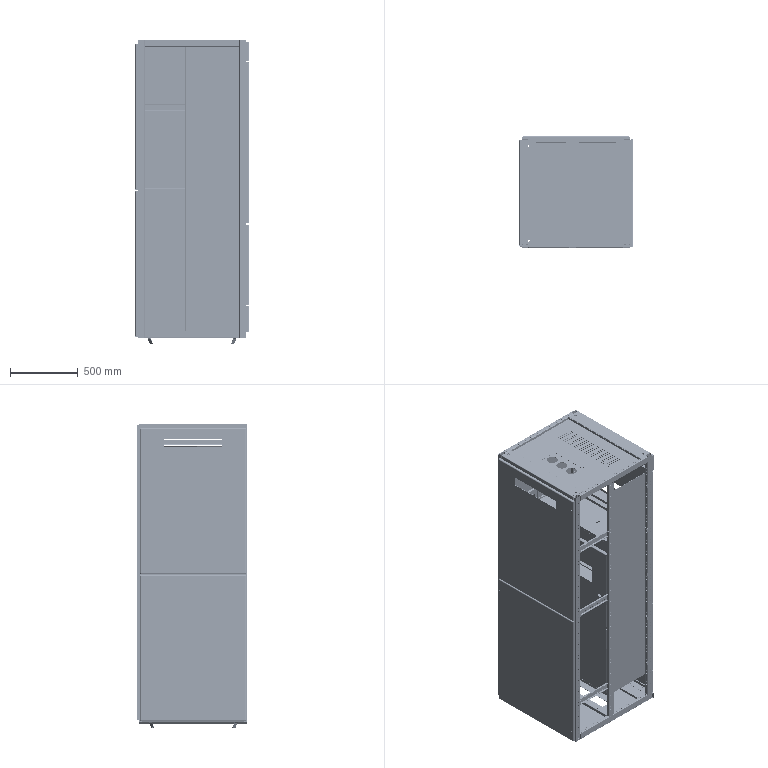Assembly | SolidWorks | mm | 93 component files | 93 solids | 13590 faces | box 836 x 818 x 2247.3 mm | volume 25225220 mm3 | cylinder 8826 | plane 4532 | cone 146 | spline 68 | torus 10 | sphere 8 | commonest cylinder face diameters 5 x6788 7 x704 6.5 x458 6 x361 2 x179 10 x64 8 x56 13 x36
Bill of materials:
Baffle(No.24) | 1 |  | Long, slender formed-sheet profile with an unequal-leg channel cross-section (a short top flange, a web, and a longer bottom flange, with rounded bends) and a regular pattern of small holes along its length.
Beam(No.10) | 2 | Plain Carbon Steel | Long lipped C-channel (a closed-looking rectangular profile with a gap in the middle of one face formed by two inturned lips), perforated along its length with rows of small holes.
Beam(No.15) | 4 |  | Long formed-sheet channel with unequal sides: a wide base, one tall side wall with a top return flange, and a short upturned lip on the other side. The wide face is perforated with a grid of small holes, there is a row of small holes along the lip, and a larger hole sits near one end.
Beam(No.20) | 6 |  | Straight channel-section beam with top and bottom flanges, a web perforated with two rows of round holes, and a folded end tab at each end carrying two larger round holes.
Beam(No.26) | 6 |  | Long angle-section member: a tall flat leg perforated with two rows of round holes, and a short perpendicular leg with tapered or chamfered ends, joined by a rounded bend.
Beam(No.30) | 1 | Plain Carbon Steel | Long, shallow tray-shaped channel: a flat base with low side walls along both long edges, and folded-up end walls, each with two small holes.
BottomCoverPlate(No.13) | 1 | Plain Carbon Steel | Rectangular flat plate with a shallow folded flange around its edges, three large round holes in a row along its centreline, and four small holes near the corners.
BottomPlate(No.14) | 1 | Plain Carbon Steel | Large rectangular sheet panel with short perimeter flanges. Two opposite flanges are interrupted by a central notch. The panel has a rectangular cutout surrounded by four small holes, a grid of elongated slots, and small holes along the flanges.
Bracket(Item49) | 4 | Plain Carbon Steel | Small formed bracket: a flat plate with two upright ears (each with a round hole) and a lower band carrying four round features with cylindrical protrusions. A perpendicular tab with two slotted holes and a bent-up central tongue projects from it.
Bracket(Item51) | 8 | Plain Carbon Steel | Small bent-strip bracket shaped like a hat or offset Z: one end leg with a round hole, a raised bridge section, and an offset outward flange with an oblong slot. All bends are rounded.
Bracket(No.11) | 4 |  | Square-based L-bracket with a rounded bend. The base has a large central round hole, two plain round holes and two countersunk-looking round features, with two short cylindrical protrusions underneath. The upright leg has two round holes, and there is a small lanced or embossed tab at the bend.
Bracket(No.35) | 8 | Plain Carbon Steel | Simple L-bracket with a rounded bend: a short leg with one larger round hole and a longer leg with two smaller round holes in line.
Brow(Item1) | 1 | Plain Carbon Steel | Long, straight bent sheet-metal profile with a constant cross-section. The section has a top flange, a long web, a rounded bend, a diagonal leg and an end flange.
ConnectingPlate(Item16) | 1 | Plain Carbon Steel | Flat rectangular plate with rounded corners and two round through-holes on its long centerline.
ConnectingPlate(No.9) | 8 | Plain Carbon Steel | Flat rectangular plate with rounded corners. It has two large round through-holes and eight smaller round holes in two rows of four.
Crossbeam(Item22) | 4 | Plain Carbon Steel | Long lipped C-channel (rounded-rectangle tube with a gap along one side) with many small round holes in rows along its length.
Block | 2 | Plain Carbon Steel | Flat rectangular plate with four chamfered corners and two round through-holes spaced along its long axis.
Crossbeam.1(Item52) | 1 | Plain Carbon Steel | Long, slender U/C-channel made of thin wall with rounded inner and outer corners and no lips.
FrontLowerDoor.2 | 1 |  | Long, thin rectangular strip plate with one large rectangular window cutout and one small square hole near one end. One long edge may have a slight bevel or rounded edge.
FrontMiddleLowerDoor | 1 |  | Flat rectangular thin panel with a large rectangular window and a narrower rectangular slot above it. It also has a pattern of tiny holes around the window and two small square holes near one edge.
hex lobular socket ctsk screws gb | 1 |  | Countersunk flat-head screw-like fastener with a hexagonal socket recess in the head and a plain cylindrical shank.
Hinge(WeldedDoor) | 5 | Plain Carbon Steel | Hinge-leaf-like flat plate with two round through-holes. One edge is rolled into an open cylindrical curl (knuckle) that runs the full length.
FrontMiddleUpperDoor | 1 |  | Flat rectangular thin panel with a row of four square cutouts along one edge region. It also has clusters of round holes above them and a small square hole near one side edge.
FrontPost | 2 | Plain Carbon Steel | Very long, slender lipped C-channel with rounded corners. A row of small perforations runs along its length.
FrontUpperDoor.2 | 1 |  | Long, thin, flat rectangular strip or plate with one small square hole near one end.
Hinge(No.46) | 1 | Plain Carbon Steel | Bent L-shaped bracket. One leg is channel-like, with raised edge rims and two round through-holes; the other leg is a flat, roughly square plate with two small embossed bumps.
LiftingRing(No.36) | 4 | Plain Carbon Steel | Flat strip with rounded ends, bent into a joggled or angled shape (a flat section, then an angled leg), with a round hole near each end.
MiddleColumn | 2 | Plain Carbon Steel | Long, slender lipped C-channel profile with a row of small perforations along its length and small notches at the ends.
Partition(No.23) | 2 | Plain Carbon Steel | Shallow rectangular tray or pan: a flat base with short upturned flanges on all four sides and a few small round holes near the corners of the long flanges.
Partition(No.29) | 1 | Plain Carbon Steel | Shallow rectangular tray or pan with perimeter flanges, several pairs of small round holes along the flanges, and four obround slots in the base.
Partition(No.50) | 1 | Plain Carbon Steel | Rectangular panel with shallow edge returns, a large rectangular cutout near the top, a single round hole, small notches at mid-height on both side edges, and small holes along the edges.
RearColumn | 2 | Plain Carbon Steel | Long, slender lipped C-channel profile with a row of small perforations along its length and small end notches.
RearLowerDoorPanel(No.28) | 1 | Plain Carbon Steel | Thin rectangular panel with slightly turned edges, a wide rectangular slot near one end, and four small holes near the corners.
RearUpperDoorPanel(No.27) | 1 | Plain Carbon Steel | Thin, plain rectangular panel with slightly turned edges and four small holes near the corners.
SidePartition(Item25) | 1 | Plain Carbon Steel | Tall, narrow thin panel with short flanges bent along both long edges, forming a shallow channel, and a row of small square holes along each flange.
SidePlate(Item17) | 1 | Plain Carbon Steel | Tall, narrow thin flat panel with a row of small holes evenly spaced along each long edge.
TopPlate(Item8) | 1 |  | Thin, flat, roughly square plate with two parallel rectangular through-slots, four larger round holes near the corners, and eight smaller round holes around the edges (two on each side).
Mates:
1. coincident | FrontPost-1 face at (398, 378, 0) dir (0, 0, 1) | assembly plane at (0, 0, 0) dir (0, 0, 1)
2. distance | assembly plane at (0, 0, 0) dir (0, 1, 0) | FrontPost-1 face at (350, 400, 0) dir (0, 1, 0)
3. distance | assembly plane at (0, 0, 0) dir (1, 0, 0) | FrontPost-1 face at (400, 400, 0) dir (1, 0, 0)
4. coincident | FrontPost-1 face at (400, 400, 0) dir (1, 0, 0) | FrontPost-2 face at (400, -400, -2200) dir (1, 0, 0)
5. coincident | FrontPost-1 face at (352, 397, 0) dir (0, 0, 1) | FrontPost-2 face at (397, -378, 0) dir (0, 0, 1)
6. distance | FrontPost-1 face at (350, 400, 0) dir (0, 1, 0) | FrontPost-2 face at (350, -400, -2200) dir (0, -1, 0)
7. coincident | FrontPost-1 face at (350, 400, 0) dir (0, 1, 0) | RearColumn-3 face at (-400, 400, 0) dir (0, 1, 0)
8. distance | RearColumn-3 face at (-400, 375, 0) dir (-1, 0, 0) | FrontPost-1 face at (400, 400, 0) dir (1, 0, 0)
9. coincident | FrontPost-1 face at (353, 377, 0) dir (0, 0, 1) | RearColumn-3 face at (-398, 397, 0) dir (0, 0, 1)
10. coincident | FrontPost-2 face at (350, -400, -2200) dir (0, -1, 0) | RearColumn-4 face at (-400, -400, -2200) dir (0, -1, 0)
11. coincident | FrontPost-2 face at (353, -398, 0) dir (0, 0, 1) | RearColumn-4 face at (-398, -378, 0) dir (0, 0, 1)
12. distance | FrontPost-2 face at (400, -400, -2200) dir (1, 0, 0) | RearColumn-4 face at (-400, -375, -2200) dir (-1, 0, 0)
13. coincident | FrontPost-1 face at (350, 400, 0) dir (0, 1, 0) | Crossbeam(Item22)-1 face at (-350, 400, -50) dir (0, 1, 0)
14. coincident | Crossbeam(Item22)-1 face at (-350, 400, 0) dir (0, 0, 1) | FrontPost-1 face at (397, 398, 0) dir (0, 0, 1)
15. coincident | FrontPost-1 face at (350, 375, 0) dir (-1, 0, 0) | Bracket(No.35)-1 face at (350, 378.5, -100) dir (1, 0, 0)
16. coincident | Crossbeam(Item22)-1 face at (-350, 375, -50) dir (0, 0, -1) | Bracket(No.35)-1 face at (350, 378.5, -50) dir (0, 0, 1)
17. concentric | Crossbeam(Item22)-1 face at (337.5, 387.5, 0) dir (0, 0, -1) r 2.5 | Bracket(No.35)-1 face at (337.5, 387.5, -52) dir (0, 0, 1) r 3.25
18. coincident | FrontPost-1 face at (350, 400, 0) dir (0, 1, 0) | Crossbeam(Item22)-3 face at (350, 400, -2150) dir (0, 1, 0)
19. coincident | FrontPost-1 face at (353, 398, -2200) dir (0, 0, -1) | Crossbeam(Item22)-3 face at (350, 400, -2200) dir (0, 0, -1)
20. coincident | FrontPost-1 face at (350, 375, 0) dir (-1, 0, 0) | Crossbeam(Item22)-3 face at (350, 398, -2197) dir (1, 0, 0)
21. coincident | RearColumn-4 face at (-400, -400, -2200) dir (0, -1, 0) | Crossbeam(Item22)-4 face at (-350, -400, -2150) dir (0, -1, 0)
22. coincident | RearColumn-4 face at (-398, -397, -2200) dir (0, 0, -1) | Crossbeam(Item22)-4 face at (-350, -400, -2200) dir (0, 0, -1)
23. coincident | RearColumn-4 face at (-350, -400, -2200) dir (1, 0, 0) | Crossbeam(Item22)-4 face at (-350, -377, -2153) dir (-1, 0, 0)
24. coincident | RearColumn-4 face at (-400, -400, -2200) dir (0, -1, 0) | Crossbeam(Item22)-2 face at (-350, -400, 0) dir (0, -1, 0)
25. coincident | RearColumn-4 face at (-352, -397, 0) dir (0, 0, 1) | Crossbeam(Item22)-2 face at (-350, -375, 0) dir (0, 0, 1)
26. coincident | RearColumn-4 face at (-350, -400, -2200) dir (1, 0, 0) | Crossbeam(Item22)-2 face at (-350, -377, -3) dir (-1, 0, 0)
27. coincident | Crossbeam(Item22)-2 face at (-350, -400, -50) dir (0, 0, -1) | Bracket(No.35)-2 face at (350, -396.5, -50) dir (0, 0, 1)
28. coincident | FrontPost-2 face at (350, -375, -2200) dir (-1, 0, 0) | Bracket(No.35)-2 face at (350, -396.5, -100) dir (1, 0, 0)
29. concentric | FrontPost-2 face at (352, -387.5, -87.5) dir (-1, 0, 0) r 2.5 | Bracket(No.35)-2 face at (350, -387.5, -87.5) dir (-1, 0, 0) r 3.25
30. coincident | RearColumn-4 face at (-350, -400, -2200) dir (1, 0, 0) | Bracket(No.35)-3 face at (-350, -378.5, -100) dir (-1, 0, 0)
31. coincident | Crossbeam(Item22)-2 face at (-350, -400, -50) dir (0, 0, -1) | Bracket(No.35)-3 face at (-350, -378.5, -50) dir (0, 0, 1)
32. concentric | RearColumn-4 face at (-352, -387.5, -87.5) dir (1, 0, 0) r 2.5 | Bracket(No.35)-3 face at (-350, -387.5, -87.5) dir (1, 0, 0) r 3.25
33. coincident | RearColumn-3 face at (-350, 400, 0) dir (1, 0, 0) | Bracket(No.35)-7 face at (-350, 396.5, -100) dir (-1, 0, 0)
34. coincident | Crossbeam(Item22)-1 face at (-350, 375, -50) dir (0, 0, -1) | Bracket(No.35)-7 face at (-350, 396.5, -50) dir (0, 0, 1)
35. concentric | RearColumn-3 face at (-352, 387.5, -87.5) dir (1, 0, 0) r 2.5 | Bracket(No.35)-7 face at (-350, 387.5, -87.5) dir (1, 0, 0) r 3.25
36. coincident | RearColumn-3 face at (-350, 400, 0) dir (1, 0, 0) | Bracket(No.35)-6 face at (-350, 378.5, -2100) dir (-1, 0, 0)
37. coincident | Crossbeam(Item22)-3 face at (350, 375, -2150) dir (0, 0, 1) | Bracket(No.35)-6 face at (-350, 378.5, -2150) dir (0, 0, -1)
38. concentric | RearColumn-3 face at (-352, 387.5, -2112.5) dir (1, 0, 0) r 2.5 | Bracket(No.35)-6 face at (-350, 387.5, -2112.5) dir (1, 0, 0) r 3.25
39. coincident | RearColumn-4 face at (-350, -400, -2200) dir (1, 0, 0) | Bracket(No.35)-5 face at (-350, -396.5, -2100) dir (-1, 0, 0)
40. coincident | Crossbeam(Item22)-4 face at (-350, -375, -2150) dir (0, 0, 1) | Bracket(No.35)-5 face at (-350, -396.5, -2150) dir (0, 0, -1)
41. concentric | RearColumn-4 face at (-352, -387.5, -2112.5) dir (1, 0, 0) r 2.5 | Bracket(No.35)-5 face at (-350, -387.5, -2112.5) dir (1, 0, 0) r 3.25
42. coincident | Crossbeam(Item22)-3 face at (350, 375, -2150) dir (0, 0, 1) | Bracket(No.35)-8 face at (350, 396.5, -2150) dir (0, 0, -1)
43. coincident | FrontPost-1 face at (350, 375, 0) dir (-1, 0, 0) | Bracket(No.35)-8 face at (350, 396.5, -2100) dir (1, 0, 0)
44. concentric | FrontPost-1 face at (352, 387.5, -2112.5) dir (-1, 0, 0) r 2.5 | Bracket(No.35)-8 face at (350, 387.5, -2112.5) dir (-1, 0, 0) r 3.25
45. coincident | Crossbeam(Item22)-4 face at (-350, -375, -2150) dir (0, 0, 1) | Bracket(No.35)-4 face at (350, -378.5, -2150) dir (0, 0, -1)
46. coincident | FrontPost-2 face at (350, -375, -2200) dir (-1, 0, 0) | Bracket(No.35)-4 face at (350, -378.5, -2100) dir (1, 0, 0)
47. concentric | FrontPost-2 face at (352, -387.5, -2112.5) dir (-1, 0, 0) r 2.5 | Bracket(No.35)-4 face at (350, -387.5, -2112.5) dir (-1, 0, 0) r 3.25
48. coincident | Crossbeam(Item22)-1 face at (-350, 400, -50) dir (0, 1, 0) | MiddleColumn-1 face at (-50, 400, -50) dir (0, 1, 0)
49. coincident | Crossbeam(Item22)-1 face at (-350, 375, -50) dir (0, 0, -1) | MiddleColumn-1 face at (-2, 378, -50) dir (0, 0, 1)
50. distance | FrontPost-1 face at (400, 400, 0) dir (1, 0, 0) | MiddleColumn-1 face at (-50, 375, -50) dir (-1, 0, 0)
51. coincident | Crossbeam(Item22)-2 face at (-350, -400, 0) dir (0, -1, 0) | MiddleColumn-2 face at (0, -400, -50) dir (0, -1, 0)
52. coincident | Crossbeam(Item22)-2 face at (-350, -400, -50) dir (0, 0, -1) | MiddleColumn-2 face at (-47, -398, -50) dir (0, 0, 1)
53. coincident | MiddleColumn-1 face at (-50, 375, -50) dir (-1, 0, 0) | MiddleColumn-2 face at (-50, -400, -50) dir (-1, 0, 0)
54. coincident | Beam(No.10)-1 face at (0, -375, -50) dir (0, 0, -1) | Crossbeam(Item22)-1 face at (-350, 375, -50) dir (0, 0, -1)
55. coincident | Crossbeam(Item22)-2 face at (-350, -375, -18.75) dir (0, 1, 0) | Beam(No.10)-1 face at (-2, -375, -47) dir (0, -1, 0)
56. coincident | MiddleColumn-2 face at (0, -375, -50) dir (1, 0, 0) | Beam(No.10)-1 face at (0, -375, -25) dir (1, 0, 0)
57. coincident | Beam(No.10)-1 face at (0, -375, -50) dir (0, 0, -1) | Bracket(No.11)-3 face at (-2.5, -329, -50) dir (0, 0, 1)
58. coincident | Crossbeam(Item22)-2 face at (-350, -375, -50) dir (0, 1, 0) | Bracket(No.11)-3 face at (-2.5, -375, -50) dir (0, -1, 0)
59. concentric | Beam(No.10)-1 face at (-37.5, -362.5, -50) dir (0, 0, 1) r 2.5 | Bracket(No.11)-3 face at (-37.5, -362.5, -50) dir (0, 0, -1) r 3.25
60. coincident | Beam(No.10)-1 face at (0, -375, -50) dir (0, 0, -1) | Bracket(No.11)-4 face at (-47.5, 329, -50) dir (0, 0, 1)
61. concentric | Beam(No.10)-1 face at (-12.5, 362.5, -50) dir (0, 0, 1) r 2.5 | Bracket(No.11)-4 face at (-12.5, 362.5, -50) dir (0, 0, -1) r 3.25
62. concentric | Beam(No.10)-1 face at (-37.5, 337.5, -50) dir (0, 0, 1) r 2.5 | Bracket(No.11)-4 face at (-37.5, 337.5, -50) dir (0, 0, -1) r 3.25
63. coincident | Crossbeam(Item22)-4 face at (-350, -400, -2200) dir (0, 0, -1) | Beam(No.15)-1 face at (300, 375, -2200) dir (0, 0, -1)
64. coincident | FrontPost-2 face at (400, -400, -2200) dir (1, 0, 0) | Beam(No.15)-1 face at (400, -375, -2150) dir (1, 0, 0)
65. coincident | FrontPost-2 face at (400, -375, -2200) dir (0, 1, 0) | Beam(No.15)-1 face at (400, -375, -2197) dir (0, -1, 0)
66. coincident | Crossbeam(Item22)-2 face at (-350, -375, 0) dir (0, 0, 1) | Beam(No.15)-2 face at (300, -375, 0) dir (0, 0, 1)
67. coincident | FrontPost-2 face at (400, -400, -2200) dir (1, 0, 0) | Beam(No.15)-2 face at (400, 375, -50) dir (1, 0, 0)
68. coincident | FrontPost-2 face at (400, -375, -2200) dir (0, 1, 0) | Beam(No.15)-2 face at (400, -375, -50) dir (0, -1, 0)
69. coincident | Crossbeam(Item22)-2 face at (-350, -375, 0) dir (0, 0, 1) | Beam(No.15)-3 face at (-300, 375, 0) dir (0, 0, 1)
70. coincident | RearColumn-4 face at (-400, -375, -2200) dir (-1, 0, 0) | Beam(No.15)-3 face at (-400, -375, -50) dir (-1, 0, 0)
71. coincident | RearColumn-3 face at (-381.25, 375, 0) dir (0, -1, 0) | Beam(No.15)-3 face at (-397, 375, -50) dir (0, 1, 0)
72. coincident | Crossbeam(Item22)-4 face at (-350, -400, -2200) dir (0, 0, -1) | Beam(No.15)-4 face at (-300, -375, -2200) dir (0, 0, -1)
73. coincident | RearColumn-4 face at (-400, -375, -2200) dir (-1, 0, 0) | Beam(No.15)-4 face at (-400, 375, -2150) dir (-1, 0, 0)
74. coincident | RearColumn-4 face at (-381.25, -375, -2200) dir (0, 1, 0) | Beam(No.15)-4 face at (-400, -375, -2197) dir (0, -1, 0)
75. coincident | FrontPost-1 face at (368.75, 375, 0) dir (0, -1, 0) | Beam(No.26)-1 face at (367.5, 375, -575) dir (0, 1, 0)
76. concentric | FrontPost-1 face at (362.5, 377, -562.5) dir (0, -1, 0) r 2.5 | Beam(No.26)-1 face at (362.5, 375, -562.5) dir (0, -1, 0) r 3.5
77. concentric | FrontPost-1 face at (362.5, 377, -537.5) dir (0, -1, 0) r 2.5 | Beam(No.26)-1 face at (362.5, 375, -537.5) dir (0, -1, 0) r 3.5
78. coincident | FrontPost-1 face at (368.75, 375, 0) dir (0, -1, 0) | Beam(No.26)-2 face at (367.5, 375, -975) dir (0, 1, 0)
79. concentric | FrontPost-1 face at (362.5, 377, -962.5) dir (0, -1, 0) r 2.5 | Beam(No.26)-2 face at (362.5, 375, -962.5) dir (0, -1, 0) r 3.5
80. concentric | FrontPost-1 face at (362.5, 377, -937.5) dir (0, -1, 0) r 2.5 | Beam(No.26)-2 face at (362.5, 375, -937.5) dir (0, -1, 0) r 3.5
81. coincident | FrontPost-1 face at (368.75, 375, 0) dir (0, -1, 0) | Beam(No.26)-3 face at (367.5, 375, -1725) dir (0, 1, 0)
82. concentric | FrontPost-1 face at (362.5, 377, -1712.5) dir (0, -1, 0) r 2.5 | Beam(No.26)-3 face at (362.5, 375, -1712.5) dir (0, -1, 0) r 3.5
83. concentric | FrontPost-1 face at (362.5, 377, -1687.5) dir (0, -1, 0) r 2.5 | Beam(No.26)-3 face at (362.5, 375, -1687.5) dir (0, -1, 0) r 3.5
84. coincident | FrontPost-2 face at (400, -375, -2200) dir (0, 1, 0) | Beam(No.26)-4 face at (-17.5, -375, -575) dir (0, -1, 0)
85. concentric | FrontPost-2 face at (362.5, -377, -562.5) dir (0, 1, 0) r 2.5 | Beam(No.26)-4 face at (362.5, -375, -562.5) dir (0, 1, 0) r 3.5
86. concentric | FrontPost-2 face at (362.5, -377, -537.5) dir (0, 1, 0) r 2.5 | Beam(No.26)-4 face at (362.5, -375, -537.5) dir (0, 1, 0) r 3.5
87. coincident | FrontPost-2 face at (368.75, -375, -2200) dir (0, 1, 0) | Beam(No.26)-6 face at (-17.5, -375, -975) dir (0, -1, 0)
88. coincident | MiddleColumn-2 face at (-50, -375, -50) dir (0, 1, 0) | Beam(No.26)-5 face at (-17.5, -375, -1725) dir (0, -1, 0)
89. concentric | FrontPost-2 face at (362.5, -377, -962.5) dir (0, 1, 0) r 2.5 | Beam(No.26)-6 face at (362.5, -375, -962.5) dir (0, 1, 0) r 3.5
90. concentric | FrontPost-2 face at (362.5, -377, -937.5) dir (0, 1, 0) r 2.5 | Beam(No.26)-6 face at (362.5, -375, -937.5) dir (0, 1, 0) r 3.5
91. concentric | FrontPost-2 face at (362.5, -377, -1712.5) dir (0, 1, 0) r 2.5 | Beam(No.26)-5 face at (362.5, -375, -1712.5) dir (0, 1, 0) r 3.5
92. concentric | FrontPost-2 face at (362.5, -377, -1687.5) dir (0, 1, 0) r 2.5 | Beam(No.26)-5 face at (362.5, -375, -1687.5) dir (0, 1, 0) r 3.5
93. coincident | Beam(No.26)-1 face at (367.5, 373, -575) dir (0, -1, 0) | Beam(No.30)-1 face at (224, 373, -570) dir (0, 1, 0)
94. concentric | Beam(No.26)-1 face at (262.5, 375, -562.5) dir (0, -1, 0) r 3.5 | Beam(No.30)-1 face at (262.5, 373, -562.5) dir (0, -1, 0) r 3.25
95. concentric | Beam(No.26)-1 face at (237.5, 375, -562.5) dir (0, -1, 0) r 3.5 | Beam(No.30)-1 face at (237.5, 373, -562.5) dir (0, -1, 0) r 3.25
96. coincident | RearColumn-4 face at (-400, -375, -2200) dir (-1, 0, 0) | Crossbeam.1(Item52)-1/Crossbeam.1(Item52)-1 face at (-400, -375, -1125) dir (-1, 0, 0)
97. concentric | RearColumn-4 face at (-362.5, -377, -1112.5) dir (0, 1, 0) r 2.5 | Crossbeam.1(Item52)-1/Block-2 face at (-362.5, -373, -1112.5) dir (0, -1, 0) r 3.25
98. coincident | RearColumn-4 face at (-350, -375, -2200) dir (0, 1, 0) | Crossbeam.1(Item52)-1/Block-2 face at (-351, -375, -1102) dir (0, -1, 0)
99. concentric | FrontPost-1 face at (362.5, 377, -587.5) dir (0, -1, 0) r 2.5 | Partition(No.29)-1 face at (362.5, 375, -587.5) dir (0, -1, 0) r 3.25
100. concentric | FrontPost-1 face at (387.5, 377, -587.5) dir (0, -1, 0) r 2.5 | Partition(No.29)-1 face at (387.5, 375, -587.5) dir (0, -1, 0) r 3.25
101. coincident | FrontPost-1 face at (368.75, 375, 0) dir (0, -1, 0) | Partition(No.29)-1 face at (397, 375, -577.5) dir (0, 1, 0)
102. coincident | Crossbeam(Item22)-4 face at (-350, -375, -2168.75) dir (0, 1, 0) | ConnectingPlate(No.9)-1 face at (395, -375, -2196) dir (0, -1, 0)
103. concentric | Crossbeam(Item22)-4 face at (312.5, -400.001, -2187.5) dir (0, 1, 0) r 2.5 | ConnectingPlate(No.9)-1 face at (312.5, -375, -2187.5) dir (0, 1, 0) r 3
104. concentric | Crossbeam(Item22)-4 face at (312.5, -400.001, -2162.5) dir (0, 1, 0) r 2.5 | ConnectingPlate(No.9)-1 face at (312.5, -375, -2162.5) dir (0, 1, 0) r 3
105. coincident | RearColumn-4 face at (-350, -375, -2200) dir (0, 1, 0) | ConnectingPlate(No.9)-2 face at (-305, -375, -2196) dir (0, -1, 0)
106. concentric | RearColumn-4 face at (-387.5, -377, -2162.5) dir (0, 1, 0) r 2.5 | ConnectingPlate(No.9)-2 face at (-387.5, -375, -2162.5) dir (0, 1, 0) r 3
107. coincident | RearColumn-4 face at (-350, -375, -2200) dir (0, 1, 0) | ConnectingPlate(No.9)-4 face at (-305, -375, -46) dir (0, -1, 0)
108. concentric | RearColumn-4 face at (-387.5, -377, -37.5) dir (0, 1, 0) r 2.5 | ConnectingPlate(No.9)-4 face at (-387.5, -375, -37.5) dir (0, 1, 0) r 3
109. concentric | RearColumn-4 face at (-387.5, -377, -12.5) dir (0, 1, 0) r 2.5 | ConnectingPlate(No.9)-4 face at (-387.5, -375, -12.5) dir (0, 1, 0) r 3
110. coincident | FrontPost-2 face at (400, -375, -2200) dir (0, 1, 0) | ConnectingPlate(No.9)-3 face at (395, -375, -46) dir (0, -1, 0)
111. concentric | FrontPost-2 face at (387.5, -377, -37.5) dir (0, 1, 0) r 2.5 | ConnectingPlate(No.9)-3 face at (387.5, -375, -37.5) dir (0, 1, 0) r 3
112. concentric | FrontPost-2 face at (387.5, -377, -12.5) dir (0, 1, 0) r 2.5 | ConnectingPlate(No.9)-3 face at (387.5, -375, -12.5) dir (0, 1, 0) r 3
113. coincident | FrontPost-1 face at (400, 375, 0) dir (0, -1, 0) | ConnectingPlate(No.9)-5 face at (395, 375, -2154) dir (0, 1, 0)
114. concentric | FrontPost-1 face at (387.5, 377, -2162.5) dir (0, -1, 0) r 2.5 | ConnectingPlate(No.9)-5 face at (387.5, 375, -2162.5) dir (0, -1, 0) r 3
115. concentric | FrontPost-1 face at (387.5, 377, -2187.5) dir (0, -1, 0) r 2.5 | ConnectingPlate(No.9)-5 face at (387.5, 375, -2187.5) dir (0, -1, 0) r 3
116. coincident | RearColumn-3 face at (-381.25, 375, 0) dir (0, -1, 0) | ConnectingPlate(No.9)-7 face at (-305, 375, -2154) dir (0, 1, 0)
117. concentric | RearColumn-3 face at (-387.5, 377, -2187.5) dir (0, -1, 0) r 2.5 | ConnectingPlate(No.9)-7 face at (-387.5, 375, -2187.5) dir (0, -1, 0) r 3
118. concentric | RearColumn-3 face at (-387.5, 377, -2162.5) dir (0, -1, 0) r 2.5 | ConnectingPlate(No.9)-7 face at (-387.5, 375, -2162.5) dir (0, -1, 0) r 3
119. coincident | FrontPost-1 face at (400, 375, 0) dir (0, -1, 0) | ConnectingPlate(No.9)-8 face at (395, 375, -4) dir (0, 1, 0)
120. concentric | FrontPost-1 face at (387.5, 377, -37.5) dir (0, -1, 0) r 2.5 | ConnectingPlate(No.9)-8 face at (387.5, 375, -37.5) dir (0, -1, 0) r 3
121. concentric | FrontPost-1 face at (387.5, 377, -12.5) dir (0, -1, 0) r 2.5 | ConnectingPlate(No.9)-8 face at (387.5, 375, -12.5) dir (0, -1, 0) r 3
122. coincident | RearColumn-3 face at (-350, 375, 0) dir (0, -1, 0) | ConnectingPlate(No.9)-6 face at (-305, 375, -4) dir (0, 1, 0)
123. concentric | RearColumn-3 face at (-387.5, 377, -37.5) dir (0, -1, 0) r 2.5 | ConnectingPlate(No.9)-6 face at (-387.5, 375, -37.5) dir (0, -1, 0) r 3
124. concentric | RearColumn-3 face at (-387.5, 377, -12.5) dir (0, -1, 0) r 2.5 | ConnectingPlate(No.9)-6 face at (-387.5, 375, -12.5) dir (0, -1, 0) r 3
125. coincident | FrontPost-1 face at (368.75, 377, 0) dir (0, 1, 0) | ConnectingPlate(Item16)-1 face at (354, 377, -2157.5) dir (0, -1, 0)
126. concentric | ConnectingPlate(Item16)-1 face at (375, 377, -2137.5) dir (0, 1, 0) r 6.5 | FrontPost-1 sketch point at (375, 400, -2137.5) dir (1, 0, 0)
127. concentric | ConnectingPlate(Item16)-1 face at (375, 377, -2087.5) dir (0, 1, 0) r 6.5 | FrontPost-1 sketch point at (375, 400, -2087.5) dir (1, 0, 0)
128. coincident | Crossbeam(Item22)-1 face at (-350, 375, 0) dir (0, -1, 0) | Bracket(Item49)-2 face at (-75, 375, -2.5) dir (0, 1, 0)
129. concentric | Crossbeam(Item22)-1 face at (12.5, 400.001, -37.5) dir (0, -1, 0) r 2.5 | Bracket(Item49)-2 face at (12.5, 375, -37.5) dir (0, -1, 0) r 3.25
130. concentric | Crossbeam(Item22)-1 face at (-62.5, 400.001, -37.5) dir (0, -1, 0) r 2.5 | Bracket(Item49)-2 face at (-62.5, 375, -37.5) dir (0, -1, 0) r 3.25
131. coincident | Crossbeam(Item22)-2 face at (-350, -375, -18.75) dir (0, 1, 0) | Bracket(Item49)-3 face at (25, -375, -2.5) dir (0, -1, 0)
132. concentric | Crossbeam(Item22)-2 face at (-62.5, -400.001, -37.5) dir (0, 1, 0) r 2.5 | Bracket(Item49)-3 face at (-62.5, -375, -37.5) dir (0, 1, 0) r 3.25
133. concentric | Crossbeam(Item22)-2 face at (12.5, -400.001, -37.5) dir (0, 1, 0) r 2.5 | Bracket(Item49)-3 face at (12.5, -375, -37.5) dir (0, 1, 0) r 3.25
134. coincident | MiddleColumn-2 face at (-18.75, -375, -50) dir (0, 1, 0) | Bracket(No.11)-2 face at (-47.5, -375, -2150) dir (0, -1, 0)
135. concentric | MiddleColumn-2 face at (-12.5, -400, -2137.5) dir (0, 1, 0) r 2.5 | Bracket(No.11)-2 face at (-12.5, -372, -2137.5) dir (0, -1, 0) r 3.25
136. concentric | MiddleColumn-2 face at (-37.5, -400, -2137.5) dir (0, 1, 0) r 2.5 | Bracket(No.11)-2 face at (-37.5, -372, -2137.5) dir (0, -1, 0) r 3.25
137. coincident | MiddleColumn-1 face at (0, 375, -50) dir (0, -1, 0) | Bracket(No.11)-1 face at (-2.5, 375, -2150) dir (0, 1, 0)
138. concentric | MiddleColumn-1 face at (-37.5, 400, -2137.5) dir (0, -1, 0) r 2.5 | Bracket(No.11)-1 face at (-37.5, 372, -2137.5) dir (0, 1, 0) r 3.25
139. concentric | MiddleColumn-1 face at (-12.5, 400, -2137.5) dir (0, -1, 0) r 2.5 | Bracket(No.11)-1 face at (-12.5, 372, -2137.5) dir (0, 1, 0) r 3.25
140. coincident | Beam(No.10)-2 face at (-50, -375, -2150) dir (0, 0, 1) | Bracket(No.11)-2 face at (-47.5, -329, -2150) dir (0, 0, -1)
141. concentric | Beam(No.10)-2 face at (-12.5, -362.5, -2150) dir (0, 0, -1) r 2.5 | Bracket(No.11)-2 face at (-12.5, -362.5, -2150) dir (0, 0, 1) r 3.25
142. concentric | Beam(No.10)-2 face at (-37.5, -337.5, -2150) dir (0, 0, -1) r 2.5 | Bracket(No.11)-2 face at (-37.5, -337.5, -2150) dir (0, 0, 1) r 3.25
143. coincident | Crossbeam(Item22)-3 face at (350, 375, -2200) dir (0, -1, 0) | Bracket(Item49)-1 face at (25, 375, -2197.5) dir (0, 1, 0)
144. concentric | Crossbeam(Item22)-3 face at (-62.5, 400.001, -2162.5) dir (0, -1, 0) r 2.5 | Bracket(Item49)-1 face at (-62.5, 375, -2162.5) dir (0, -1, 0) r 3.25
145. concentric | Crossbeam(Item22)-3 face at (12.5, 400.001, -2162.5) dir (0, -1, 0) r 2.5 | Bracket(Item49)-1 face at (12.5, 375, -2162.5) dir (0, -1, 0) r 3.25
146. coincident | Crossbeam(Item22)-4 face at (-350, -375, -2200) dir (0, 1, 0) | Bracket(Item49)-4 face at (-75, -375, -2197.5) dir (0, -1, 0)
147. concentric | Crossbeam(Item22)-4 face at (-62.5, -400.001, -2162.5) dir (0, 1, 0) r 2.5 | Bracket(Item49)-4 face at (-62.5, -375, -2162.5) dir (0, 1, 0) r 3.25
148. concentric | Crossbeam(Item22)-4 face at (12.5, -400.001, -2162.5) dir (0, 1, 0) r 2.5 | Bracket(Item49)-4 face at (12.5, -375, -2162.5) dir (0, 1, 0) r 3.25
149. coincident | RearColumn-3 face at (-381.25, 375, 0) dir (0, -1, 0) | Bracket(Item51)-1 face at (-400, 375, -122.5) dir (0, 1, 0)
150. coincident | RearColumn-3 face at (-400, 375, 0) dir (-1, 0, 0) | Bracket(Item51)-1 face at (-400, 390, -122.5) dir (1, 0, 0)
151. coincident | RearColumn-3 face at (-381.25, 375, 0) dir (0, -1, 0) | Bracket(Item51)-4 face at (-400, 375, -1222.5) dir (0, 1, 0)
152. coincident | RearColumn-3 face at (-400, 375, 0) dir (-1, 0, 0) | Bracket(Item51)-4 face at (-400, 390, -1222.5) dir (1, 0, 0)
153. coincident | RearColumn-3 face at (-381.25, 375, 0) dir (0, -1, 0) | Bracket(Item51)-2 face at (-400, 375, -2122.5) dir (0, 1, 0)
154. coincident | RearColumn-3 face at (-400, 375, 0) dir (-1, 0, 0) | Bracket(Item51)-2 face at (-400, 390, -2122.5) dir (1, 0, 0)
155. coincident | RearColumn-3 face at (-381.25, 375, 0) dir (0, -1, 0) | Bracket(Item51)-3 face at (-400, 375, -1022.5) dir (0, 1, 0)
156. coincident | RearColumn-3 face at (-400, 375, 0) dir (-1, 0, 0) | Bracket(Item51)-3 face at (-400, 390, -1022.5) dir (1, 0, 0)
157. coincident | RearColumn-4 face at (-400, -375, -2200) dir (-1, 0, 0) | RearLowerDoorPanel(No.28)-1 face at (-400, 392, -1110) dir (1, 0, 0)
158. coincident | RearColumn-3 face at (-400, 375, 0) dir (-1, 0, 0) | RearUpperDoorPanel(No.27)-1 face at (-400, -392, -1115) dir (1, 0, 0)
159. distance | RearLowerDoorPanel(No.28)-1 face at (-400, -392, -1110) dir (0, 0, -1) | RearUpperDoorPanel(No.27)-1 face at (-400, 392, -1115) dir (0, 0, 1)
160. coincident | RearLowerDoorPanel(No.28)-1 face at (-416, 392, -30) dir (0, 1, 0) | RearUpperDoorPanel(No.27)-1 face at (-416, 392, -1115) dir (0, 1, 0)
161. distance | RearUpperDoorPanel(No.27)-1 face at (-416, 392, -1115) dir (0, 1, 0) | RearColumn-3 face at (-400, 400, 0) dir (0, 1, 0)
162. distance | RearUpperDoorPanel(No.27)-1 face at (-400, 392, -1115) dir (0, 0, 1) | Crossbeam.1(Item52)-1/Crossbeam.1(Item52)-1 face at (-375, -375, -1125) dir (0, 0, -1)
163. concentric | RearColumn-3 face at (-387.5, 377, -2112.5) dir (0, -1, 0) r 2.5 | Bracket(Item51)-2 sketch segment at (-387.5, 373, -2112.5) dir (0, -1, 0) r 2.285
164. concentric | RearColumn-3 face at (-387.5, 377, -1212.5) dir (0, -1, 0) r 2.5 | Bracket(Item51)-4 sketch segment at (-387.5, 373, -1212.5) dir (0, -1, 0) r 2.285
165. concentric | RearColumn-3 face at (-387.5, 377, -1012.5) dir (0, -1, 0) r 2.5 | Bracket(Item51)-3 sketch segment at (-387.5, 373, -1012.5) dir (0, -1, 0) r 2.285
166. concentric | RearColumn-3 face at (-387.5, 377, -112.5) dir (0, -1, 0) r 2.5 | Bracket(Item51)-1 sketch segment at (-387.5, 373, -112.5) dir (0, -1, 0) r 2.285
167. coincident | RearColumn-4 face at (-381.25, -375, -2200) dir (0, 1, 0) | Bracket(Item51)-5 face at (-400, -375, -102.5) dir (0, -1, 0)
168. coincident | RearColumn-4 face at (-400, -375, -2200) dir (-1, 0, 0) | Bracket(Item51)-5 face at (-400, -390, -102.5) dir (1, 0, 0)
169. coincident | Bracket(Item51)-1 face at (-402, 386, -122.5) dir (0, 0, -1) | Bracket(Item51)-5 face at (-404, -388, -122.5) dir (0, 0, -1)
170. coincident | RearColumn-4 face at (-381.25, -375, -2200) dir (0, 1, 0) | Bracket(Item51)-7 face at (-400, -375, -2102.5) dir (0, -1, 0)
171. coincident | RearColumn-4 face at (-381.25, -375, -2200) dir (0, 1, 0) | Bracket(Item51)-6 face at (-400, -375, -1002.5) dir (0, -1, 0)
172. coincident | RearColumn-4 face at (-381.25, -375, -2200) dir (0, 1, 0) | Bracket(Item51)-8 face at (-400, -375, -1202.5) dir (0, -1, 0)
173. coincident | RearColumn-4 face at (-400, -375, -2200) dir (-1, 0, 0) | Bracket(Item51)-7 face at (-400, -390, -2102.5) dir (1, 0, 0)
174. coincident | RearColumn-4 face at (-400, -375, -2200) dir (-1, 0, 0) | Bracket(Item51)-6 face at (-400, -390, -1002.5) dir (1, 0, 0)
175. coincident | RearColumn-4 face at (-400, -375, -2200) dir (-1, 0, 0) | Bracket(Item51)-8 face at (-400, -390, -1202.5) dir (1, 0, 0)
176. coincident | Bracket(Item51)-4 face at (-402, 386, -1222.5) dir (0, 0, -1) | Bracket(Item51)-8 face at (-413, -386, -1222.5) dir (0, 0, -1)
177. coincident | Bracket(Item51)-3 face at (-402, 386, -1022.5) dir (0, 0, -1) | Bracket(Item51)-6 face at (-413, -386, -1022.5) dir (0, 0, -1)
178. coincident | Bracket(Item51)-2 face at (-402, 386, -2122.5) dir (0, 0, -1) | Bracket(Item51)-7 face at (-413, -386, -2122.5) dir (0, 0, -1)
179. coincident | RearColumn-3 face at (-400, 400, 0) dir (0, 1, 0) | SidePlate(Item17)-1 face at (-395, 400, -10) dir (0, -1, 0)
180. distance | Crossbeam(Item22)-3 face at (350, 400, -2200) dir (0, 0, -1) | SidePlate(Item17)-1 face at (-395, 400, -2190) dir (0, 0, -1)
181. distance | FrontPost-1 face at (400, 400, 0) dir (1, 0, 0) | SidePlate(Item17)-1 face at (395, 400, -2190) dir (1, 0, 0)
182. coincident | FrontPost-1 face at (400, 375, 0) dir (0, -1, 0) | Partition(No.23)-1 face at (400, 375, -1952.5) dir (0, 1, 0)
183. coincident | FrontPost-1 face at (368.75, 375, 0) dir (0, -1, 0) | Partition(No.23)-2 face at (400, 375, -1352.5) dir (0, 1, 0)
184. coincident | Beam(No.15)-1 face at (397, 375, -2150) dir (0, 0, 1) | Baffle(No.24)-1 face at (400, -375, -2150) dir (0, 0, -1)
185. coincident | Beam(No.15)-1 face at (400, -375, -2150) dir (1, 0, 0) | Baffle(No.24)-1 face at (400, -375, -2121.5) dir (1, 0, 0)
186. coincident | FrontPost-1 face at (400, 375, 0) dir (0, -1, 0) | Baffle(No.24)-1 face at (397, 375, -2147) dir (0, 1, 0)
187. concentric | Beam(No.15)-4 face at (-350, -350, -2200) dir (0, 0, 1) r 10 | TopPlate(Item8)-1 face at (-350, -350, -2202) dir (0, 0, 1) r 8.5
188. concentric | Beam(No.15)-4 face at (-350, 350, -2200) dir (0, 0, 1) r 10 | TopPlate(Item8)-1 face at (-350, 350, -2202) dir (0, 0, 1) r 8.5
189. coincident | Beam(No.15)-4 face at (-300, -375, -2200) dir (0, 0, -1) | TopPlate(Item8)-1 face at (-400, 400, -2200) dir (0, 0, 1)
190. coincident | TopPlate(Item8)-1 face at (-400, 400, -2202) dir (0, 0, -1) | LiftingRing(No.36)-1 face at (-370.153, -348.939, -2202) dir (0, 0, 1)
191. concentric | TopPlate(Item8)-1 face at (-350, -350, -2202) dir (0, 0, 1) r 8.5 | LiftingRing(No.36)-1 face at (-350, -350, -2204) dir (0, 0, 1) r 7.5
192. angle | TopPlate(Item8)-1 face at (400, -400, -2202) dir (0, -1, 0) | LiftingRing(No.36)-1 face at (-304.268, -325.481, -2205.5) dir (0.7071, -0.7071, 0)
193. coincident | TopPlate(Item8)-1 face at (-400, 400, -2202) dir (0, 0, -1) | LiftingRing(No.36)-2 face at (348.939, -370.153, -2202) dir (0, 0, 1)
194. coincident | TopPlate(Item8)-1 face at (-400, 400, -2202) dir (0, 0, -1) | LiftingRing(No.36)-4 face at (370.153, 348.939, -2202) dir (0, 0, 1)
195. coincident | TopPlate(Item8)-1 face at (-400, 400, -2202) dir (0, 0, -1) | LiftingRing(No.36)-3 face at (-348.939, 370.153, -2202) dir (0, 0, 1)
196. concentric | TopPlate(Item8)-1 face at (350, -350, -2202) dir (0, 0, 1) r 8.5 | LiftingRing(No.36)-2 face at (350, -350, -2204) dir (0, 0, 1) r 7.5
197. angle | LiftingRing(No.36)-2 face at (325.481, -304.268, -2205.5) dir (0.7071, 0.7071, 0) | TopPlate(Item8)-1 face at (375, -400, -2202) dir (1, 0, 0)
198. concentric | TopPlate(Item8)-1 face at (350, 350, -2202) dir (0, 0, 1) r 8.5 | LiftingRing(No.36)-4 face at (350, 350, -2204) dir (0, 0, 1) r 7.5
199. angle | LiftingRing(No.36)-4 face at (329.767, 308.554, -2209) dir (0.7071, -0.7071, 0) | TopPlate(Item8)-1 face at (375, -400, -2202) dir (1, 0, 0)
200. concentric | TopPlate(Item8)-1 face at (-350, 350, -2202) dir (0, 0, 1) r 8.5 | LiftingRing(No.36)-3 face at (-350, 350, -2204) dir (0, 0, 1) r 7.5
201. angle | LiftingRing(No.36)-3 face at (-308.554, 329.767, -2209) dir (0.7071, 0.7071, 0) | TopPlate(Item8)-1 face at (400, 400, -2202) dir (0, 1, 0)
202. coincident | Partition(No.23)-1 face at (-50, -375, -1952.5) dir (0, -1, 0) | SidePartition(Item25)-3 face at (350, -375, -1972.5) dir (0, 1, 0)
203. coincident | FrontPost-2 face at (350, -375, -2200) dir (-1, 0, 0) | SidePartition(Item25)-3 face at (350, -399, -1972.5) dir (1, 0, 0)
204. coincident | Partition(No.23)-1 face at (-50, 375, -1972.5) dir (0, 0, -1) | SidePartition(Item25)-3 face at (0, -375, -1972.5) dir (0, 0, -1)
205. coincident | Beam(No.15)-2 face at (300, 375, -3) dir (-1, 0, 0) | BottomPlate(No.14)-1 face at (300, -375, -3.5) dir (1, 0, 0)
206. concentric | Beam(No.15)-3 face at (-303, 212.5, -12.5) dir (1, 0, 0) r 2.5 | BottomPlate(No.14)-1 face at (300, 212.5, -12.5) dir (-1, 0, 0) r 3.25
207. concentric | Beam(No.15)-3 face at (-303, -212.5, -12.5) dir (1, 0, 0) r 2.5 | BottomPlate(No.14)-1 face at (300, -212.5, -12.5) dir (-1, 0, 0) r 3.25
208. coincident | BottomPlate(No.14)-1 face at (-300, 375, -21.5) dir (0, 0, -1) | BottomCoverPlate(No.13)-1 face at (-50, 170, -21.5) dir (0, 0, 1)
209. concentric | BottomPlate(No.14)-1 face at (-230, 140, -19.5) dir (0, 0, -1) r 2.5 | BottomCoverPlate(No.13)-1 face at (-230, 140, -29.5) dir (0, 0, -1) r 3.25
210. concentric | BottomPlate(No.14)-1 face at (-230, -140, -19.5) dir (0, 0, -1) r 2.5 | BottomCoverPlate(No.13)-1 face at (-230, -140, -29.5) dir (0, 0, -1) r 3.25
211. coincident | FrontPost-1 face at (400, 400, 0) dir (1, 0, 0) | FrontUpperDoor.2-1 face at (400, 395, -2155.5) dir (-1, 0, 0)
212. distance | FrontUpperDoor.2-1 face at (416, 395, -1968.5) dir (0, 1, 0) | FrontPost-1 face at (350, 400, 0) dir (0, 1, 0)
213. coincident | FrontPost-2 face at (400, -400, -2200) dir (1, 0, 0) | FrontMiddleUpperDoor-1/FrontMiddleUpperDoor-1 face at (400, -395, -1955.5) dir (-1, 0, 0)
214. distance | FrontUpperDoor.2-1 face at (416, -395, -1965.5) dir (0, 0, 1) | FrontMiddleUpperDoor-1/FrontMiddleUpperDoor-1 face at (416, 395, -1955.5) dir (0, 0, -1)
215. distance | FrontMiddleUpperDoor-1/FrontMiddleUpperDoor-1 face at (416, -395, -1955.5) dir (0, -1, 0) | FrontPost-2 face at (350, -400, -2200) dir (0, -1, 0)
216. coincident | FrontPost-1 face at (400, 400, 0) dir (1, 0, 0) | FrontMiddleLowerDoor-1/FrontMiddleLowerDoor-1 face at (400, 395, -1355.5) dir (-1, 0, 0)
217. distance | FrontMiddleLowerDoor-1/FrontMiddleLowerDoor-1 face at (416, 395, -1355.5) dir (0, 0, -1) | FrontMiddleUpperDoor-1/FrontMiddleUpperDoor-1 face at (416, -395, -1365.5) dir (0, 0, 1)
218. distance | FrontMiddleLowerDoor-1/FrontMiddleLowerDoor-1 face at (416, -395, -1355.5) dir (0, -1, 0) | FrontPost-2 face at (350, -400, -2200) dir (0, -1, 0)
219. coincident | FrontPost-2 face at (400, -400, -2200) dir (1, 0, 0) | FrontLowerDoor.2-1 face at (400, -396, -155.5) dir (-1, 0, 0)
220. distance | FrontMiddleLowerDoor-1/FrontMiddleLowerDoor-1 face at (416, -395, -165.5) dir (0, 0, 1) | FrontLowerDoor.2-1 face at (416, 394, -155.5) dir (0, 0, -1)
221. distance | FrontLowerDoor.2-1 face at (416, -396, -155.5) dir (0, -1, 0) | FrontPost-2 face at (350, -400, -2200) dir (0, -1, 0)
222. concentric | RearColumn-4 face at (-387.5, -377, -2187.5) dir (0, 1, 0) r 2.5 | ConnectingPlate(No.9)-2 face at (-387.5, -375, -2187.5) dir (0, 1, 0) r 3
223. coincident | FrontPost-1 face at (400, 375, 0) dir (0, -1, 0) | Hinge(No.46)-1 face at (400.986, 375, -2109.5) dir (0, 1, 0)
224. concentric | FrontPost-1 face at (362.5, 377, -2087.5) dir (0, -1, 0) r 2.5 | Hinge(No.46)-1 face at (362.5, 375, -2087.5) dir (0, -1, 0) r 3
225. concentric | FrontPost-1 face at (387.5, 377, -2087.5) dir (0, -1, 0) r 2.5 | Hinge(No.46)-1 face at (387.5, 375, -2087.5) dir (0, -1, 0) r 3
226. coincident | Beam(No.15)-1 face at (300, 375, -2200) dir (0, 0, -1) | Brow(Item1)-1 face at (400, -398, -2200) dir (0, 0, 1)
227. coincident | Beam(No.15)-1 face at (400, -375, -2150) dir (1, 0, 0) | Brow(Item1)-1 face at (400, -398, -2166.5) dir (-1, 0, 0)
228. distance | Brow(Item1)-1 face at (399.352, 398, -2203) dir (0, 1, 0) | TopPlate(Item8)-1 face at (400, 400, -2202) dir (0, 1, 0)
229. distance | Brow(Item1)-1 face at (400, -398, -2165) dir (0, 0, 1) | FrontUpperDoor.2-1 face at (416, 395, -2155.5) dir (0, 0, -1)
230. concentric | FrontPost-1 face at (387.5, 377, -1962.5) dir (0, -1, 0) r 2.5 | Partition(No.23)-1 face at (387.5, 375, -1962.5) dir (0, -1, 0) r 3.25
231. concentric | FrontPost-1 face at (387.5, 377, -1362.5) dir (0, -1, 0) r 2.5 | Partition(No.23)-2 face at (387.5, 375, -1362.5) dir (0, -1, 0) r 3.25
232. concentric | FrontPost-1 face at (362.5, 377, -1362.5) dir (0, -1, 0) r 2.5 | Partition(No.23)-2 face at (362.5, 375, -1362.5) dir (0, -1, 0) r 3.25
233. concentric | MiddleColumn-2 face at (-50, -387.5, -512.5) dir (1, 0, 0) r 2.5 | Beam(No.20)-1 face at (-350, -387.5, -512.5) dir (1, 0, 0) r 3.5
234. concentric | MiddleColumn-2 face at (-50, -387.5, -487.5) dir (1, 0, 0) r 2.5 | Beam(No.20)-1 face at (-350, -387.5, -487.5) dir (1, 0, 0) r 3.5
235. coincident | MiddleColumn-2 face at (-50, -400, -50) dir (-1, 0, 0) | Beam(No.20)-1 face at (-50, -377, -478) dir (1, 0, 0)
236. concentric | MiddleColumn-2 face at (-50, -387.5, -1087.5) dir (1, 0, 0) r 2.5 | Beam(No.20)-2 face at (-350, -387.5, -1087.5) dir (1, 0, 0) r 3.5
237. concentric | MiddleColumn-2 face at (-50, -387.5, -1062.5) dir (1, 0, 0) r 2.5 | Beam(No.20)-2 face at (-350, -387.5, -1062.5) dir (1, 0, 0) r 3.5
238. coincident | MiddleColumn-2 face at (-50, -400, -50) dir (-1, 0, 0) | Beam(No.20)-2 face at (-50, -377, -1053) dir (1, 0, 0)
239. concentric | MiddleColumn-2 face at (-50, -387.5, -1887.5) dir (1, 0, 0) r 2.5 | Beam(No.20)-3 face at (-350, -387.5, -1887.5) dir (1, 0, 0) r 3.5
240. coincident | MiddleColumn-2 face at (-50, -400, -50) dir (-1, 0, 0) | Beam(No.20)-3 face at (-50, -377, -1853) dir (1, 0, 0)
241. concentric | MiddleColumn-1 face at (0, 387.5, -512.5) dir (-1, 0, 0) r 2.5 | Beam(No.20)-4 face at (-350, 387.5, -512.5) dir (1, 0, 0) r 3.5
242. concentric | MiddleColumn-1 face at (0, 387.5, -487.5) dir (-1, 0, 0) r 2.5 | Beam(No.20)-4 face at (-350, 387.5, -487.5) dir (1, 0, 0) r 3.5
243. coincident | MiddleColumn-1 face at (-50, 375, -50) dir (-1, 0, 0) | Beam(No.20)-4 face at (-50, 377, -522) dir (1, 0, 0)
244. concentric | MiddleColumn-1 face at (0, 387.5, -1087.5) dir (-1, 0, 0) r 2.5 | Beam(No.20)-5 face at (-350, 387.5, -1087.5) dir (1, 0, 0) r 3.5
245. concentric | MiddleColumn-1 face at (0, 387.5, -1062.5) dir (-1, 0, 0) r 2.5 | Beam(No.20)-5 face at (-350, 387.5, -1062.5) dir (1, 0, 0) r 3.5
246. coincident | MiddleColumn-1 face at (-50, 375, -50) dir (-1, 0, 0) | Beam(No.20)-5 face at (-50, 377, -1097) dir (1, 0, 0)
247. concentric | MiddleColumn-1 face at (0, 387.5, -1887.5) dir (-1, 0, 0) r 2.5 | Beam(No.20)-6 face at (-350, 387.5, -1887.5) dir (1, 0, 0) r 3.5
248. concentric | MiddleColumn-1 face at (0, 387.5, -1862.5) dir (-1, 0, 0) r 2.5 | Beam(No.20)-6 face at (-350, 387.5, -1862.5) dir (1, 0, 0) r 3.5
249. coincident | MiddleColumn-1 face at (-50, 375, -50) dir (-1, 0, 0) | Beam(No.20)-6 face at (-50, 377, -1897) dir (1, 0, 0)
250. coincident | Partition(No.23)-2 face at (-50, -372, -1370.5) dir (-1, 0, 0) | Partition(No.50)-1 face at (-50, 375, -1952.5) dir (1, 0, 0)
251. coincident | Partition(No.50)-1 edge at (-27, 372.929, -1952.5) dir (0, -1, 0) | Partition(No.23)-1 face at (-50, 372, -1952.5) dir (0, 0, 1)
252. coincident | MiddleColumn-1 face at (-31.25, 375, -50) dir (0, -1, 0) | Partition(No.50)-1 face at (-27, 375, -1952.5) dir (0, 1, 0)
253. coordinate | Crossbeam.1(Item52)-1 sketch point at (0, 0, 0) dir (1, 0, 0) | Crossbeam.1(Item52) sketch point at (0, 0, 0) dir (1, 0, 0)
254. coincident | Crossbeam.1(Item52)-1 face at (-12.5, -2, 750) dir (0, -1, 0) | Block-1 face at (-10.5, -2, 0) dir (0, 1, 0)
255. coincident | Crossbeam.1(Item52)-1 face at (10.5, -3, 0) dir (0, 0, -1) | Block-1 face at (10.5, -49, 0) dir (0, 0, -1)
256. coincident | Crossbeam.1(Item52)-1 plane at (0, 0, 0) dir (1, 0, 0) | Block-1 plane at (0, -25.5, 2) dir (1, 0, 0)
257. coincident | Block-1 face at (-10.5, -2, 0) dir (-1, 0, 0) | Block-2 face at (-10.5, -2, 748) dir (-1, 0, 0)
258. coincident | Crossbeam.1(Item52)-1 face at (-12.5, -2, 750) dir (0, -1, 0) | Block-2 face at (-10.5, -2, 748) dir (0, 1, 0)
259. coincident | Crossbeam.1(Item52)-1 face at (-10.5, -3, 750) dir (0, 0, 1) | Block-2 face at (10.5, -49, 750) dir (0, 0, 1)
260. coordinate | FrontMiddleLowerDoor-1 sketch point at (0, 0, 0) dir (1, 0, 0) | FrontMiddleLowerDoor sketch point at (0, 0, 0) dir (1, 0, 0)
261. coincident | FrontMiddleLowerDoor-1 face at (595, 395, -2) dir (0, 0, -1) | Hinge(WeldedDoor)-1 face at (17.5, 388.5, -2) dir (0, 0, 1)
262. tangent | FrontMiddleLowerDoor-1 face at (-592, 393, -2) dir (0, -1, 0) | Hinge(WeldedDoor)-1 face at (17.5, 388.5, -6.5) dir (-1, 0, 0) r 4.5
263. coincident | FrontMiddleLowerDoor-1 plane at (0, 0, 0) dir (1, 0, 0) | Hinge(WeldedDoor)-1 plane at (0, 388.5, -6.5) dir (1, 0, 0)
264. coincident | FrontMiddleLowerDoor-1 face at (595, 395, -2) dir (0, 0, -1) | hex lobular socket ctsk screws gb-2 face at (-525, 319, -2) dir (0, 0, 1)
265. concentric | FrontMiddleLowerDoor-1 sketch segment at (-525, 319, -2) dir (0, 0, -1) r 5 | hex lobular socket ctsk screws gb-2 face at (-525, 319, -36.6) dir (0, 0, 1) r 3
266. coordinate | FrontMiddleUpperDoor-1 sketch point at (0, 0, 0) dir (1, 0, 0) | FrontMiddleUpperDoor sketch point at (0, 0, 0) dir (1, 0, 0)
267. coincident | FrontMiddleUpperDoor-1 face at (295, 395, -2) dir (0, 0, -1) | Hinge(WeldedDoor)-1 face at (205, 388.5, -2) dir (0, 0, 1)
268. distance | Hinge(WeldedDoor)-1 face at (205, 388.5, -6.5) dir (1, 0, 0) | FrontMiddleUpperDoor-1 face at (295, 395, -2) dir (1, 0, 0)
269. tangent | FrontMiddleUpperDoor-1 face at (-292, 393, -2) dir (0, -1, 0) | Hinge(WeldedDoor)-1 face at (205, 388.5, -6.5) dir (-1, 0, 0) r 4.5